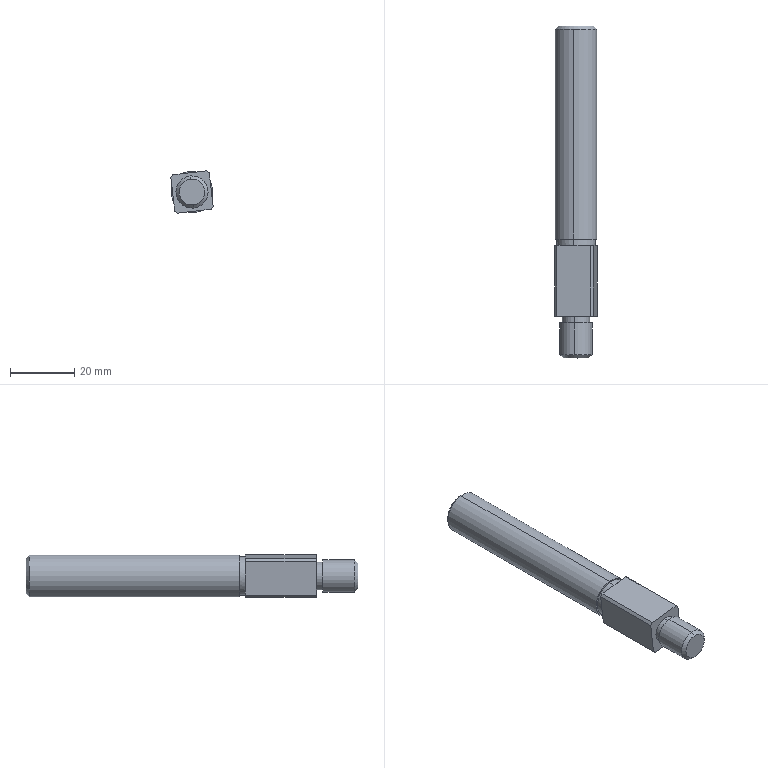Component | SolidWorks | 23-1 | 1 solid | 29 faces | box 13.13 x 103 x 13.13 mm | volume 13082 mm3 | plane 13 | cylinder 12 | cone 4 | commonest cylinder face diameters 16 x4 10 x2 8.5 x2 12 x2 13 x2
STEP:
#1=COLOUR_RGB('',0.7922,0.8196,0.9333);
#2=FILL_AREA_STYLE_COLOUR('',#1);
#3=FILL_AREA_STYLE('',(#2));
#4=SURFACE_STYLE_FILL_AREA(#3);
#5=SURFACE_SIDE_STYLE('',(#4));
#6=SURFACE_STYLE_USAGE(.BOTH.,#5);
#7=PRESENTATION_STYLE_ASSIGNMENT((#6));
#8=CARTESIAN_POINT('',(-5.893,13.153,28.394));
#9=VERTEX_POINT('',#8);
#10=CARTESIAN_POINT('',(-5.843,13.153,27.964));
#11=VERTEX_POINT('',#10);
#12=CARTESIAN_POINT('',(-5.868,13.153,28.179));
#13=DIRECTION('',(0.,1.,-0.));
#14=DIRECTION('',(0.114,0.,-0.9935));
#15=AXIS2_PLACEMENT_3D('',#12,#13,#14);
#16=CIRCLE('',#15,0.2165);
#17=EDGE_CURVE('',#9,#11,#16,.T.);
#18=ORIENTED_EDGE('',*,*,#17,.F.);
#19=CARTESIAN_POINT('',(-5.897,13.114,28.433));
#20=VERTEX_POINT('',#19);
#21=CARTESIAN_POINT('',(-5.897,13.114,28.433));
#22=DIRECTION('',(-0.08059,-0.7071,0.7025));
#23=VECTOR('',#22,39.37);
#24=LINE('',#21,#23);
#25=EDGE_CURVE('',#9,#20,#24,.T.);
#26=ORIENTED_EDGE('',*,*,#25,.T.);
#27=CARTESIAN_POINT('',(-5.839,13.114,27.925));
#28=VERTEX_POINT('',#27);
#29=CARTESIAN_POINT('',(-5.868,13.114,28.179));
#30=DIRECTION('',(-0.,-1.,0.));
#31=DIRECTION('',(0.114,0.,-0.9935));
#32=AXIS2_PLACEMENT_3D('',#29,#30,#31);
#33=CIRCLE('',#32,0.2559);
#34=EDGE_CURVE('',#28,#20,#33,.T.);
#35=ORIENTED_EDGE('',*,*,#34,.F.);
#36=CARTESIAN_POINT('',(-5.839,13.114,27.925));
#37=DIRECTION('',(0.08059,-0.7071,-0.7025));
#38=VECTOR('',#37,39.37);
#39=LINE('',#36,#38);
#40=EDGE_CURVE('',#11,#28,#39,.T.);
#41=ORIENTED_EDGE('',*,*,#40,.F.);
#42=EDGE_LOOP('',(#18,#26,#35,#41));
#43=FACE_OUTER_BOUND('',#42,.T.);
#44=CARTESIAN_POINT('',(-5.868,13.114,28.179));
#45=DIRECTION('',(-0.,-1.,0.));
#46=DIRECTION('',(0.114,0.,-0.9935));
#47=AXIS2_PLACEMENT_3D('',#44,#45,#46);
#48=CONICAL_SURFACE('',#47,0.2559,0.7854);
#49=ADVANCED_FACE('',(#43),#48,.T.);
#50=CARTESIAN_POINT('',(-5.85,9.098,28.023));
#51=VERTEX_POINT('',#50);
#52=CARTESIAN_POINT('',(-5.886,9.098,28.336));
#53=VERTEX_POINT('',#52);
#54=CARTESIAN_POINT('',(-5.868,9.098,28.179));
#55=DIRECTION('',(-0.,-1.,0.));
#56=DIRECTION('',(-0.114,0.,0.9935));
#57=AXIS2_PLACEMENT_3D('',#54,#55,#56);
#58=CIRCLE('',#57,0.1575);
#59=EDGE_CURVE('',#51,#53,#58,.T.);
#60=ORIENTED_EDGE('',*,*,#59,.F.);
#61=CARTESIAN_POINT('',(-5.845,9.137,27.984));
#62=VERTEX_POINT('',#61);
#63=CARTESIAN_POINT('',(-5.85,9.098,28.023));
#64=DIRECTION('',(0.08059,0.7071,-0.7025));
#65=VECTOR('',#64,39.37);
#66=LINE('',#63,#65);
#67=EDGE_CURVE('',#51,#62,#66,.T.);
#68=ORIENTED_EDGE('',*,*,#67,.T.);
#69=CARTESIAN_POINT('',(-5.89,9.137,28.375));
#70=VERTEX_POINT('',#69);
#71=CARTESIAN_POINT('',(-5.868,9.137,28.179));
#72=DIRECTION('',(0.,1.,-0.));
#73=DIRECTION('',(-0.114,0.,0.9935));
#74=AXIS2_PLACEMENT_3D('',#71,#72,#73);
#75=CIRCLE('',#74,0.1969);
#76=EDGE_CURVE('',#70,#62,#75,.T.);
#77=ORIENTED_EDGE('',*,*,#76,.F.);
#78=CARTESIAN_POINT('',(-5.886,9.098,28.336));
#79=DIRECTION('',(-0.08059,0.7071,0.7025));
#80=VECTOR('',#79,39.37);
#81=LINE('',#78,#80);
#82=EDGE_CURVE('',#53,#70,#81,.T.);
#83=ORIENTED_EDGE('',*,*,#82,.F.);
#84=EDGE_LOOP('',(#60,#68,#77,#83));
#85=FACE_OUTER_BOUND('',#84,.T.);
#86=CARTESIAN_POINT('',(-5.868,9.098,28.179));
#87=DIRECTION('',(0.,1.,-0.));
#88=DIRECTION('',(-0.114,0.,0.9935));
#89=AXIS2_PLACEMENT_3D('',#86,#87,#88);
#90=CONICAL_SURFACE('',#89,0.1575,0.7854);
#91=ADVANCED_FACE('',(#85),#90,.T.);
#92=CARTESIAN_POINT('',(-5.845,9.527,27.984));
#93=VERTEX_POINT('',#92);
#94=CARTESIAN_POINT('',(-5.89,9.527,28.375));
#95=VERTEX_POINT('',#94);
#96=CARTESIAN_POINT('',(-5.868,9.527,28.179));
#97=DIRECTION('',(-0.,-1.,0.));
#98=DIRECTION('',(0.114,0.,-0.9935));
#99=AXIS2_PLACEMENT_3D('',#96,#97,#98);
#100=CIRCLE('',#99,0.1969);
#101=EDGE_CURVE('',#93,#95,#100,.T.);
#102=ORIENTED_EDGE('',*,*,#101,.T.);
#103=CARTESIAN_POINT('',(-5.89,9.098,28.375));
#104=DIRECTION('',(-0.,-1.,0.));
#105=VECTOR('',#104,39.37);
#106=LINE('',#103,#105);
#107=EDGE_CURVE('',#95,#70,#106,.T.);
#108=ORIENTED_EDGE('',*,*,#107,.T.);
#109=ORIENTED_EDGE('',*,*,#76,.T.);
#110=CARTESIAN_POINT('',(-5.845,9.098,27.984));
#111=DIRECTION('',(-0.,-1.,0.));
#112=VECTOR('',#111,39.37);
#113=LINE('',#110,#112);
#114=EDGE_CURVE('',#93,#62,#113,.T.);
#115=ORIENTED_EDGE('',*,*,#114,.F.);
#116=EDGE_LOOP('',(#102,#108,#109,#115));
#117=FACE_OUTER_BOUND('',#116,.T.);
#118=CARTESIAN_POINT('',(-5.868,9.098,28.179));
#119=DIRECTION('',(-0.,-1.,0.));
#120=DIRECTION('',(0.114,0.,-0.9935));
#121=AXIS2_PLACEMENT_3D('',#118,#119,#120);
#122=CYLINDRICAL_SURFACE('',#121,0.1969);
#123=ADVANCED_FACE('',(#117),#122,.T.);
#124=CARTESIAN_POINT('',(-5.849,9.606,28.013));
#125=VERTEX_POINT('',#124);
#126=CARTESIAN_POINT('',(-5.887,9.606,28.345));
#127=VERTEX_POINT('',#126);
#128=CARTESIAN_POINT('',(-5.868,9.606,28.179));
#129=DIRECTION('',(-0.,-1.,0.));
#130=DIRECTION('',(0.114,0.,-0.9935));
#131=AXIS2_PLACEMENT_3D('',#128,#129,#130);
#132=CIRCLE('',#131,0.1673);
#133=EDGE_CURVE('',#125,#127,#132,.T.);
#134=ORIENTED_EDGE('',*,*,#133,.T.);
#135=CARTESIAN_POINT('',(-5.887,9.527,28.345));
#136=VERTEX_POINT('',#135);
#137=CARTESIAN_POINT('',(-5.887,9.098,28.345));
#138=DIRECTION('',(-0.,-1.,0.));
#139=VECTOR('',#138,39.37);
#140=LINE('',#137,#139);
#141=EDGE_CURVE('',#127,#136,#140,.T.);
#142=ORIENTED_EDGE('',*,*,#141,.T.);
#143=CARTESIAN_POINT('',(-5.849,9.527,28.013));
#144=VERTEX_POINT('',#143);
#145=CARTESIAN_POINT('',(-5.868,9.527,28.179));
#146=DIRECTION('',(-0.,-1.,0.));
#147=DIRECTION('',(0.114,0.,-0.9935));
#148=AXIS2_PLACEMENT_3D('',#145,#146,#147);
#149=CIRCLE('',#148,0.1673);
#150=EDGE_CURVE('',#144,#136,#149,.T.);
#151=ORIENTED_EDGE('',*,*,#150,.F.);
#152=CARTESIAN_POINT('',(-5.849,9.098,28.013));
#153=DIRECTION('',(-0.,-1.,0.));
#154=VECTOR('',#153,39.37);
#155=LINE('',#152,#154);
#156=EDGE_CURVE('',#125,#144,#155,.T.);
#157=ORIENTED_EDGE('',*,*,#156,.F.);
#158=EDGE_LOOP('',(#134,#142,#151,#157));
#159=FACE_OUTER_BOUND('',#158,.T.);
#160=CARTESIAN_POINT('',(-5.868,9.098,28.179));
#161=DIRECTION('',(-0.,-1.,0.));
#162=DIRECTION('',(0.114,0.,-0.9935));
#163=AXIS2_PLACEMENT_3D('',#160,#161,#162);
#164=CYLINDRICAL_SURFACE('',#163,0.1673);
#165=ADVANCED_FACE('',(#159),#164,.T.);
#166=CARTESIAN_POINT('',(-5.841,10.551,27.944));
#167=VERTEX_POINT('',#166);
#168=CARTESIAN_POINT('',(-5.895,10.551,28.414));
#169=VERTEX_POINT('',#168);
#170=CARTESIAN_POINT('',(-5.868,10.551,28.179));
#171=DIRECTION('',(-0.,-1.,0.));
#172=DIRECTION('',(0.114,0.,-0.9935));
#173=AXIS2_PLACEMENT_3D('',#170,#171,#172);
#174=CIRCLE('',#173,0.2362);
#175=EDGE_CURVE('',#167,#169,#174,.T.);
#176=ORIENTED_EDGE('',*,*,#175,.T.);
#177=CARTESIAN_POINT('',(-5.895,10.472,28.414));
#178=VERTEX_POINT('',#177);
#179=CARTESIAN_POINT('',(-5.895,9.098,28.414));
#180=DIRECTION('',(-0.,-1.,0.));
#181=VECTOR('',#180,39.37);
#182=LINE('',#179,#181);
#183=EDGE_CURVE('',#169,#178,#182,.T.);
#184=ORIENTED_EDGE('',*,*,#183,.T.);
#185=CARTESIAN_POINT('',(-5.633,10.472,28.206));
#186=VERTEX_POINT('',#185);
#187=CARTESIAN_POINT('',(-5.868,10.472,28.179));
#188=DIRECTION('',(-0.,-1.,0.));
#189=DIRECTION('',(0.114,0.,-0.9935));
#190=AXIS2_PLACEMENT_3D('',#187,#188,#189);
#191=CIRCLE('',#190,0.2362);
#192=EDGE_CURVE('',#186,#178,#191,.T.);
#193=ORIENTED_EDGE('',*,*,#192,.F.);
#194=CARTESIAN_POINT('',(-5.841,10.472,27.944));
#195=VERTEX_POINT('',#194);
#196=CARTESIAN_POINT('',(-5.868,10.472,28.179));
#197=DIRECTION('',(-0.,-1.,0.));
#198=DIRECTION('',(0.114,0.,-0.9935));
#199=AXIS2_PLACEMENT_3D('',#196,#197,#198);
#200=CIRCLE('',#199,0.2362);
#201=EDGE_CURVE('',#195,#186,#200,.T.);
#202=ORIENTED_EDGE('',*,*,#201,.F.);
#203=CARTESIAN_POINT('',(-5.841,9.098,27.944));
#204=DIRECTION('',(-0.,-1.,0.));
#205=VECTOR('',#204,39.37);
#206=LINE('',#203,#205);
#207=EDGE_CURVE('',#167,#195,#206,.T.);
#208=ORIENTED_EDGE('',*,*,#207,.F.);
#209=EDGE_LOOP('',(#176,#184,#193,#202,#208));
#210=FACE_OUTER_BOUND('',#209,.T.);
#211=CARTESIAN_POINT('',(-5.868,9.098,28.179));
#212=DIRECTION('',(-0.,-1.,0.));
#213=DIRECTION('',(0.114,0.,-0.9935));
#214=AXIS2_PLACEMENT_3D('',#211,#212,#213);
#215=CYLINDRICAL_SURFACE('',#214,0.2362);
#216=ADVANCED_FACE('',(#210),#215,.T.);
#217=ORIENTED_EDGE('',*,*,#34,.T.);
#218=CARTESIAN_POINT('',(-5.897,10.551,28.433));
#219=VERTEX_POINT('',#218);
#220=CARTESIAN_POINT('',(-5.897,9.098,28.433));
#221=DIRECTION('',(-0.,-1.,0.));
#222=VECTOR('',#221,39.37);
#223=LINE('',#220,#222);
#224=EDGE_CURVE('',#20,#219,#223,.T.);
#225=ORIENTED_EDGE('',*,*,#224,.T.);
#226=CARTESIAN_POINT('',(-5.839,10.551,27.925));
#227=VERTEX_POINT('',#226);
#228=CARTESIAN_POINT('',(-5.868,10.551,28.179));
#229=DIRECTION('',(-0.,-1.,0.));
#230=DIRECTION('',(0.114,0.,-0.9935));
#231=AXIS2_PLACEMENT_3D('',#228,#229,#230);
#232=CIRCLE('',#231,0.2559);
#233=EDGE_CURVE('',#227,#219,#232,.T.);
#234=ORIENTED_EDGE('',*,*,#233,.F.);
#235=CARTESIAN_POINT('',(-5.839,9.098,27.925));
#236=DIRECTION('',(-0.,-1.,0.));
#237=VECTOR('',#236,39.37);
#238=LINE('',#235,#237);
#239=EDGE_CURVE('',#28,#227,#238,.T.);
#240=ORIENTED_EDGE('',*,*,#239,.F.);
#241=EDGE_LOOP('',(#217,#225,#234,#240));
#242=FACE_OUTER_BOUND('',#241,.T.);
#243=CARTESIAN_POINT('',(-5.868,9.098,28.179));
#244=DIRECTION('',(-0.,-1.,0.));
#245=DIRECTION('',(0.114,0.,-0.9935));
#246=AXIS2_PLACEMENT_3D('',#243,#244,#245);
#247=CYLINDRICAL_SURFACE('',#246,0.2559);
#248=ADVANCED_FACE('',(#242),#247,.T.);
#249=CARTESIAN_POINT('',(-6.102,10.472,28.39));
#250=VERTEX_POINT('',#249);
#251=CARTESIAN_POINT('',(-6.126,10.472,28.359));
#252=VERTEX_POINT('',#251);
#253=CARTESIAN_POINT('',(-5.868,10.472,28.179));
#254=DIRECTION('',(-0.,-1.,0.));
#255=DIRECTION('',(0.114,0.,-0.9935));
#256=AXIS2_PLACEMENT_3D('',#253,#254,#255);
#257=CIRCLE('',#256,0.315);
#258=EDGE_CURVE('',#250,#252,#257,.T.);
#259=ORIENTED_EDGE('',*,*,#258,.F.);
#260=CARTESIAN_POINT('',(-5.895,10.472,28.414));
#261=DIRECTION('',(0.9935,-0.,0.114));
#262=VECTOR('',#261,39.37);
#263=LINE('',#260,#262);
#264=EDGE_CURVE('',#250,#178,#263,.T.);
#265=ORIENTED_EDGE('',*,*,#264,.T.);
#266=CARTESIAN_POINT('',(-6.103,10.472,28.152));
#267=VERTEX_POINT('',#266);
#268=CARTESIAN_POINT('',(-5.868,10.472,28.179));
#269=DIRECTION('',(-0.,-1.,0.));
#270=DIRECTION('',(0.114,0.,-0.9935));
#271=AXIS2_PLACEMENT_3D('',#268,#269,#270);
#272=CIRCLE('',#271,0.2362);
#273=EDGE_CURVE('',#178,#267,#272,.T.);
#274=ORIENTED_EDGE('',*,*,#273,.T.);
#275=CARTESIAN_POINT('',(-6.103,10.472,28.152));
#276=DIRECTION('',(0.114,-0.,-0.9935));
#277=VECTOR('',#276,39.37);
#278=LINE('',#275,#277);
#279=EDGE_CURVE('',#252,#267,#278,.T.);
#280=ORIENTED_EDGE('',*,*,#279,.F.);
#281=EDGE_LOOP('',(#259,#265,#274,#280));
#282=FACE_OUTER_BOUND('',#281,.T.);
#283=CARTESIAN_POINT('',(-5.895,10.472,28.414));
#284=DIRECTION('',(-0.,-1.,0.));
#285=DIRECTION('',(0.114,-0.,-0.9935));
#286=AXIS2_PLACEMENT_3D('',#283,#284,#285);
#287=PLANE('',#286);
#288=ADVANCED_FACE('',(#282),#287,.F.);
#289=ORIENTED_EDGE('',*,*,#192,.T.);
#290=CARTESIAN_POINT('',(-5.688,10.472,28.438));
#291=VERTEX_POINT('',#290);
#292=CARTESIAN_POINT('',(-5.895,10.472,28.414));
#293=DIRECTION('',(0.9935,-0.,0.114));
#294=VECTOR('',#293,39.37);
#295=LINE('',#292,#294);
#296=EDGE_CURVE('',#178,#291,#295,.T.);
#297=ORIENTED_EDGE('',*,*,#296,.T.);
#298=CARTESIAN_POINT('',(-5.657,10.472,28.413));
#299=VERTEX_POINT('',#298);
#300=CARTESIAN_POINT('',(-5.868,10.472,28.179));
#301=DIRECTION('',(-0.,-1.,0.));
#302=DIRECTION('',(0.114,0.,-0.9935));
#303=AXIS2_PLACEMENT_3D('',#300,#301,#302);
#304=CIRCLE('',#303,0.315);
#305=EDGE_CURVE('',#299,#291,#304,.T.);
#306=ORIENTED_EDGE('',*,*,#305,.F.);
#307=CARTESIAN_POINT('',(-5.633,10.472,28.206));
#308=DIRECTION('',(0.114,-0.,-0.9935));
#309=VECTOR('',#308,39.37);
#310=LINE('',#307,#309);
#311=EDGE_CURVE('',#299,#186,#310,.T.);
#312=ORIENTED_EDGE('',*,*,#311,.T.);
#313=EDGE_LOOP('',(#289,#297,#306,#312));
#314=FACE_OUTER_BOUND('',#313,.T.);
#315=CARTESIAN_POINT('',(-5.895,10.472,28.414));
#316=DIRECTION('',(-0.,-1.,0.));
#317=DIRECTION('',(0.114,-0.,-0.9935));
#318=AXIS2_PLACEMENT_3D('',#315,#316,#317);
#319=PLANE('',#318);
#320=ADVANCED_FACE('',(#314),#319,.F.);
#321=CARTESIAN_POINT('',(-6.048,10.472,27.921));
#322=VERTEX_POINT('',#321);
#323=CARTESIAN_POINT('',(-5.841,10.472,27.944));
#324=DIRECTION('',(0.9935,-0.,0.114));
#325=VECTOR('',#324,39.37);
#326=LINE('',#323,#325);
#327=EDGE_CURVE('',#322,#195,#326,.T.);
#328=ORIENTED_EDGE('',*,*,#327,.F.);
#329=CARTESIAN_POINT('',(-6.079,10.472,27.945));
#330=VERTEX_POINT('',#329);
#331=CARTESIAN_POINT('',(-5.868,10.472,28.179));
#332=DIRECTION('',(-0.,-1.,0.));
#333=DIRECTION('',(0.114,0.,-0.9935));
#334=AXIS2_PLACEMENT_3D('',#331,#332,#333);
#335=CIRCLE('',#334,0.315);
#336=EDGE_CURVE('',#330,#322,#335,.T.);
#337=ORIENTED_EDGE('',*,*,#336,.F.);
#338=CARTESIAN_POINT('',(-6.103,10.472,28.152));
#339=DIRECTION('',(0.114,-0.,-0.9935));
#340=VECTOR('',#339,39.37);
#341=LINE('',#338,#340);
#342=EDGE_CURVE('',#267,#330,#341,.T.);
#343=ORIENTED_EDGE('',*,*,#342,.F.);
#344=CARTESIAN_POINT('',(-5.868,10.472,28.179));
#345=DIRECTION('',(-0.,-1.,0.));
#346=DIRECTION('',(0.114,0.,-0.9935));
#347=AXIS2_PLACEMENT_3D('',#344,#345,#346);
#348=CIRCLE('',#347,0.2362);
#349=EDGE_CURVE('',#267,#195,#348,.T.);
#350=ORIENTED_EDGE('',*,*,#349,.T.);
#351=EDGE_LOOP('',(#328,#337,#343,#350));
#352=FACE_OUTER_BOUND('',#351,.T.);
#353=CARTESIAN_POINT('',(-5.895,10.472,28.414));
#354=DIRECTION('',(-0.,-1.,0.));
#355=DIRECTION('',(0.114,-0.,-0.9935));
#356=AXIS2_PLACEMENT_3D('',#353,#354,#355);
#357=PLANE('',#356);
#358=ADVANCED_FACE('',(#352),#357,.F.);
#359=ORIENTED_EDGE('',*,*,#201,.T.);
#360=CARTESIAN_POINT('',(-5.609,10.472,27.999));
#361=VERTEX_POINT('',#360);
#362=CARTESIAN_POINT('',(-5.633,10.472,28.206));
#363=DIRECTION('',(0.114,-0.,-0.9935));
#364=VECTOR('',#363,39.37);
#365=LINE('',#362,#364);
#366=EDGE_CURVE('',#186,#361,#365,.T.);
#367=ORIENTED_EDGE('',*,*,#366,.T.);
#368=CARTESIAN_POINT('',(-5.634,10.472,27.968));
#369=VERTEX_POINT('',#368);
#370=CARTESIAN_POINT('',(-5.868,10.472,28.179));
#371=DIRECTION('',(-0.,-1.,0.));
#372=DIRECTION('',(0.114,0.,-0.9935));
#373=AXIS2_PLACEMENT_3D('',#370,#371,#372);
#374=CIRCLE('',#373,0.315);
#375=EDGE_CURVE('',#369,#361,#374,.T.);
#376=ORIENTED_EDGE('',*,*,#375,.F.);
#377=CARTESIAN_POINT('',(-5.841,10.472,27.944));
#378=DIRECTION('',(0.9935,-0.,0.114));
#379=VECTOR('',#378,39.37);
#380=LINE('',#377,#379);
#381=EDGE_CURVE('',#195,#369,#380,.T.);
#382=ORIENTED_EDGE('',*,*,#381,.F.);
#383=EDGE_LOOP('',(#359,#367,#376,#382));
#384=FACE_OUTER_BOUND('',#383,.T.);
#385=CARTESIAN_POINT('',(-5.895,10.472,28.414));
#386=DIRECTION('',(-0.,-1.,0.));
#387=DIRECTION('',(0.114,-0.,-0.9935));
#388=AXIS2_PLACEMENT_3D('',#385,#386,#387);
#389=PLANE('',#388);
#390=ADVANCED_FACE('',(#384),#389,.F.);
#391=ORIENTED_EDGE('',*,*,#305,.T.);
#392=CARTESIAN_POINT('',(-5.688,9.606,28.438));
#393=VERTEX_POINT('',#392);
#394=CARTESIAN_POINT('',(-5.688,10.472,28.438));
#395=DIRECTION('',(-0.,-1.,0.));
#396=VECTOR('',#395,39.37);
#397=LINE('',#394,#396);
#398=EDGE_CURVE('',#291,#393,#397,.T.);
#399=ORIENTED_EDGE('',*,*,#398,.T.);
#400=CARTESIAN_POINT('',(-5.657,9.606,28.413));
#401=VERTEX_POINT('',#400);
#402=CARTESIAN_POINT('',(-5.868,9.606,28.179));
#403=DIRECTION('',(-0.,-1.,0.));
#404=DIRECTION('',(0.114,0.,-0.9935));
#405=AXIS2_PLACEMENT_3D('',#402,#403,#404);
#406=CIRCLE('',#405,0.315);
#407=EDGE_CURVE('',#401,#393,#406,.T.);
#408=ORIENTED_EDGE('',*,*,#407,.F.);
#409=CARTESIAN_POINT('',(-5.657,10.472,28.413));
#410=DIRECTION('',(-0.,-1.,0.));
#411=VECTOR('',#410,39.37);
#412=LINE('',#409,#411);
#413=EDGE_CURVE('',#299,#401,#412,.T.);
#414=ORIENTED_EDGE('',*,*,#413,.F.);
#415=EDGE_LOOP('',(#391,#399,#408,#414));
#416=FACE_OUTER_BOUND('',#415,.T.);
#417=CARTESIAN_POINT('',(-5.868,9.098,28.179));
#418=DIRECTION('',(-0.,-1.,0.));
#419=DIRECTION('',(0.114,0.,-0.9935));
#420=AXIS2_PLACEMENT_3D('',#417,#418,#419);
#421=CYLINDRICAL_SURFACE('',#420,0.315);
#422=ADVANCED_FACE('',(#416),#421,.T.);
#423=ORIENTED_EDGE('',*,*,#375,.T.);
#424=CARTESIAN_POINT('',(-5.609,9.606,27.999));
#425=VERTEX_POINT('',#424);
#426=CARTESIAN_POINT('',(-5.609,10.472,27.999));
#427=DIRECTION('',(-0.,-1.,0.));
#428=VECTOR('',#427,39.37);
#429=LINE('',#426,#428);
#430=EDGE_CURVE('',#361,#425,#429,.T.);
#431=ORIENTED_EDGE('',*,*,#430,.T.);
#432=CARTESIAN_POINT('',(-5.634,9.606,27.968));
#433=VERTEX_POINT('',#432);
#434=CARTESIAN_POINT('',(-5.868,9.606,28.179));
#435=DIRECTION('',(-0.,-1.,0.));
#436=DIRECTION('',(0.114,0.,-0.9935));
#437=AXIS2_PLACEMENT_3D('',#434,#435,#436);
#438=CIRCLE('',#437,0.315);
#439=EDGE_CURVE('',#433,#425,#438,.T.);
#440=ORIENTED_EDGE('',*,*,#439,.F.);
#441=CARTESIAN_POINT('',(-5.634,10.472,27.968));
#442=DIRECTION('',(-0.,-1.,0.));
#443=VECTOR('',#442,39.37);
#444=LINE('',#441,#443);
#445=EDGE_CURVE('',#369,#433,#444,.T.);
#446=ORIENTED_EDGE('',*,*,#445,.F.);
#447=EDGE_LOOP('',(#423,#431,#440,#446));
#448=FACE_OUTER_BOUND('',#447,.T.);
#449=CARTESIAN_POINT('',(-5.868,9.098,28.179));
#450=DIRECTION('',(-0.,-1.,0.));
#451=DIRECTION('',(0.114,0.,-0.9935));
#452=AXIS2_PLACEMENT_3D('',#449,#450,#451);
#453=CYLINDRICAL_SURFACE('',#452,0.315);
#454=ADVANCED_FACE('',(#448),#453,.T.);
#455=CARTESIAN_POINT('',(-6.102,9.606,28.39));
#456=VERTEX_POINT('',#455);
#457=CARTESIAN_POINT('',(-6.126,9.606,28.359));
#458=VERTEX_POINT('',#457);
#459=CARTESIAN_POINT('',(-5.868,9.606,28.179));
#460=DIRECTION('',(-0.,-1.,0.));
#461=DIRECTION('',(0.114,0.,-0.9935));
#462=AXIS2_PLACEMENT_3D('',#459,#460,#461);
#463=CIRCLE('',#462,0.315);
#464=EDGE_CURVE('',#456,#458,#463,.T.);
#465=ORIENTED_EDGE('',*,*,#464,.F.);
#466=CARTESIAN_POINT('',(-6.102,10.472,28.39));
#467=DIRECTION('',(-0.,-1.,0.));
#468=VECTOR('',#467,39.37);
#469=LINE('',#466,#468);
#470=EDGE_CURVE('',#250,#456,#469,.T.);
#471=ORIENTED_EDGE('',*,*,#470,.F.);
#472=ORIENTED_EDGE('',*,*,#258,.T.);
#473=CARTESIAN_POINT('',(-6.126,10.472,28.359));
#474=DIRECTION('',(-0.,-1.,0.));
#475=VECTOR('',#474,39.37);
#476=LINE('',#473,#475);
#477=EDGE_CURVE('',#252,#458,#476,.T.);
#478=ORIENTED_EDGE('',*,*,#477,.T.);
#479=EDGE_LOOP('',(#465,#471,#472,#478));
#480=FACE_OUTER_BOUND('',#479,.T.);
#481=CARTESIAN_POINT('',(-5.868,9.098,28.179));
#482=DIRECTION('',(-0.,-1.,0.));
#483=DIRECTION('',(0.114,0.,-0.9935));
#484=AXIS2_PLACEMENT_3D('',#481,#482,#483);
#485=CYLINDRICAL_SURFACE('',#484,0.315);
#486=ADVANCED_FACE('',(#480),#485,.T.);
#487=CARTESIAN_POINT('',(-6.048,9.606,27.921));
#488=VERTEX_POINT('',#487);
#489=CARTESIAN_POINT('',(-6.048,10.472,27.921));
#490=DIRECTION('',(-0.,-1.,0.));
#491=VECTOR('',#490,39.37);
#492=LINE('',#489,#491);
#493=EDGE_CURVE('',#322,#488,#492,.T.);
#494=ORIENTED_EDGE('',*,*,#493,.T.);
#495=CARTESIAN_POINT('',(-6.079,9.606,27.945));
#496=VERTEX_POINT('',#495);
#497=CARTESIAN_POINT('',(-5.868,9.606,28.179));
#498=DIRECTION('',(-0.,-1.,0.));
#499=DIRECTION('',(0.114,0.,-0.9935));
#500=AXIS2_PLACEMENT_3D('',#497,#498,#499);
#501=CIRCLE('',#500,0.315);
#502=EDGE_CURVE('',#496,#488,#501,.T.);
#503=ORIENTED_EDGE('',*,*,#502,.F.);
#504=CARTESIAN_POINT('',(-6.079,10.472,27.945));
#505=DIRECTION('',(-0.,-1.,0.));
#506=VECTOR('',#505,39.37);
#507=LINE('',#504,#506);
#508=EDGE_CURVE('',#330,#496,#507,.T.);
#509=ORIENTED_EDGE('',*,*,#508,.F.);
#510=ORIENTED_EDGE('',*,*,#336,.T.);
#511=EDGE_LOOP('',(#494,#503,#509,#510));
#512=FACE_OUTER_BOUND('',#511,.T.);
#513=CARTESIAN_POINT('',(-5.868,9.098,28.179));
#514=DIRECTION('',(-0.,-1.,0.));
#515=DIRECTION('',(0.114,0.,-0.9935));
#516=AXIS2_PLACEMENT_3D('',#513,#514,#515);
#517=CYLINDRICAL_SURFACE('',#516,0.315);
#518=ADVANCED_FACE('',(#512),#517,.T.);
#519=ORIENTED_EDGE('',*,*,#133,.F.);
#520=CARTESIAN_POINT('',(-5.868,9.606,28.179));
#521=DIRECTION('',(-0.,-1.,0.));
#522=DIRECTION('',(0.114,0.,-0.9935));
#523=AXIS2_PLACEMENT_3D('',#520,#521,#522);
#524=CIRCLE('',#523,0.1673);
#525=EDGE_CURVE('',#127,#125,#524,.T.);
#526=ORIENTED_EDGE('',*,*,#525,.F.);
#527=EDGE_LOOP('',(#519,#526));
#528=FACE_BOUND('',#527,.T.);
#529=ORIENTED_EDGE('',*,*,#407,.T.);
#530=CARTESIAN_POINT('',(-5.895,9.606,28.414));
#531=DIRECTION('',(0.9935,-0.,0.114));
#532=VECTOR('',#531,39.37);
#533=LINE('',#530,#532);
#534=EDGE_CURVE('',#456,#393,#533,.T.);
#535=ORIENTED_EDGE('',*,*,#534,.F.);
#536=ORIENTED_EDGE('',*,*,#464,.T.);
#537=CARTESIAN_POINT('',(-6.103,9.606,28.152));
#538=DIRECTION('',(0.114,-0.,-0.9935));
#539=VECTOR('',#538,39.37);
#540=LINE('',#537,#539);
#541=EDGE_CURVE('',#458,#496,#540,.T.);
#542=ORIENTED_EDGE('',*,*,#541,.T.);
#543=ORIENTED_EDGE('',*,*,#502,.T.);
#544=CARTESIAN_POINT('',(-5.841,9.606,27.944));
#545=DIRECTION('',(0.9935,-0.,0.114));
#546=VECTOR('',#545,39.37);
#547=LINE('',#544,#546);
#548=EDGE_CURVE('',#488,#433,#547,.T.);
#549=ORIENTED_EDGE('',*,*,#548,.T.);
#550=ORIENTED_EDGE('',*,*,#439,.T.);
#551=CARTESIAN_POINT('',(-5.633,9.606,28.206));
#552=DIRECTION('',(0.114,-0.,-0.9935));
#553=VECTOR('',#552,39.37);
#554=LINE('',#551,#553);
#555=EDGE_CURVE('',#401,#425,#554,.T.);
#556=ORIENTED_EDGE('',*,*,#555,.F.);
#557=EDGE_LOOP('',(#529,#535,#536,#542,#543,#549,#550,#556));
#558=FACE_OUTER_BOUND('',#557,.T.);
#559=CARTESIAN_POINT('',(-5.904,9.606,28.492));
#560=DIRECTION('',(0.,1.,-0.));
#561=DIRECTION('',(-0.114,0.,0.9935));
#562=AXIS2_PLACEMENT_3D('',#559,#560,#561);
#563=PLANE('',#562);
#564=ADVANCED_FACE('',(#528,#558),#563,.F.);
#565=CARTESIAN_POINT('',(-5.868,9.098,28.179));
#566=DIRECTION('',(-0.,-1.,0.));
#567=DIRECTION('',(-0.114,0.,0.9935));
#568=AXIS2_PLACEMENT_3D('',#565,#566,#567);
#569=CIRCLE('',#568,0.1575);
#570=EDGE_CURVE('',#53,#51,#569,.T.);
#571=ORIENTED_EDGE('',*,*,#570,.T.);
#572=ORIENTED_EDGE('',*,*,#59,.T.);
#573=EDGE_LOOP('',(#571,#572));
#574=FACE_OUTER_BOUND('',#573,.T.);
#575=CARTESIAN_POINT('',(-5.89,9.098,28.375));
#576=DIRECTION('',(0.,1.,-0.));
#577=DIRECTION('',(-0.114,0.,0.9935));
#578=AXIS2_PLACEMENT_3D('',#575,#576,#577);
#579=PLANE('',#578);
#580=ADVANCED_FACE('',(#574),#579,.F.);
#581=CARTESIAN_POINT('',(-5.868,13.153,28.179));
#582=DIRECTION('',(0.,1.,-0.));
#583=DIRECTION('',(0.114,0.,-0.9935));
#584=AXIS2_PLACEMENT_3D('',#581,#582,#583);
#585=CIRCLE('',#584,0.2165);
#586=EDGE_CURVE('',#11,#9,#585,.T.);
#587=ORIENTED_EDGE('',*,*,#586,.T.);
#588=ORIENTED_EDGE('',*,*,#17,.T.);
#589=EDGE_LOOP('',(#587,#588));
#590=FACE_OUTER_BOUND('',#589,.T.);
#591=CARTESIAN_POINT('',(-5.868,13.153,28.179));
#592=DIRECTION('',(-0.,-1.,0.));
#593=DIRECTION('',(0.114,-0.,-0.9935));
#594=AXIS2_PLACEMENT_3D('',#591,#592,#593);
#595=PLANE('',#594);
#596=ADVANCED_FACE('',(#590),#595,.F.);
#597=ORIENTED_EDGE('',*,*,#224,.F.);
#598=CARTESIAN_POINT('',(-5.868,13.114,28.179));
#599=DIRECTION('',(-0.,-1.,0.));
#600=DIRECTION('',(0.114,0.,-0.9935));
#601=AXIS2_PLACEMENT_3D('',#598,#599,#600);
#602=CIRCLE('',#601,0.2559);
#603=EDGE_CURVE('',#20,#28,#602,.T.);
#604=ORIENTED_EDGE('',*,*,#603,.T.);
#605=ORIENTED_EDGE('',*,*,#239,.T.);
#606=CARTESIAN_POINT('',(-5.868,10.551,28.179));
#607=DIRECTION('',(-0.,-1.,0.));
#608=DIRECTION('',(0.114,0.,-0.9935));
#609=AXIS2_PLACEMENT_3D('',#606,#607,#608);
#610=CIRCLE('',#609,0.2559);
#611=EDGE_CURVE('',#219,#227,#610,.T.);
#612=ORIENTED_EDGE('',*,*,#611,.F.);
#613=EDGE_LOOP('',(#597,#604,#605,#612));
#614=FACE_OUTER_BOUND('',#613,.T.);
#615=CARTESIAN_POINT('',(-5.868,9.098,28.179));
#616=DIRECTION('',(-0.,-1.,0.));
#617=DIRECTION('',(0.114,0.,-0.9935));
#618=AXIS2_PLACEMENT_3D('',#615,#616,#617);
#619=CYLINDRICAL_SURFACE('',#618,0.2559);
#620=ADVANCED_FACE('',(#614),#619,.T.);
#621=ORIENTED_EDGE('',*,*,#175,.F.);
#622=CARTESIAN_POINT('',(-5.868,10.551,28.179));
#623=DIRECTION('',(-0.,-1.,0.));
#624=DIRECTION('',(0.114,0.,-0.9935));
#625=AXIS2_PLACEMENT_3D('',#622,#623,#624);
#626=CIRCLE('',#625,0.2362);
#627=EDGE_CURVE('',#169,#167,#626,.T.);
#628=ORIENTED_EDGE('',*,*,#627,.F.);
#629=EDGE_LOOP('',(#621,#628));
#630=FACE_BOUND('',#629,.T.);
#631=ORIENTED_EDGE('',*,*,#233,.T.);
#632=ORIENTED_EDGE('',*,*,#611,.T.);
#633=EDGE_LOOP('',(#631,#632));
#634=FACE_OUTER_BOUND('',#633,.T.);
#635=CARTESIAN_POINT('',(-5.897,10.551,28.433));
#636=DIRECTION('',(0.,1.,-0.));
#637=DIRECTION('',(-0.114,0.,0.9935));
#638=AXIS2_PLACEMENT_3D('',#635,#636,#637);
#639=PLANE('',#638);
#640=ADVANCED_FACE('',(#630,#634),#639,.F.);
#641=ORIENTED_EDGE('',*,*,#183,.F.);
#642=ORIENTED_EDGE('',*,*,#627,.T.);
#643=ORIENTED_EDGE('',*,*,#207,.T.);
#644=ORIENTED_EDGE('',*,*,#349,.F.);
#645=ORIENTED_EDGE('',*,*,#273,.F.);
#646=EDGE_LOOP('',(#641,#642,#643,#644,#645));
#647=FACE_OUTER_BOUND('',#646,.T.);
#648=CARTESIAN_POINT('',(-5.868,9.098,28.179));
#649=DIRECTION('',(-0.,-1.,0.));
#650=DIRECTION('',(0.114,0.,-0.9935));
#651=AXIS2_PLACEMENT_3D('',#648,#649,#650);
#652=CYLINDRICAL_SURFACE('',#651,0.2362);
#653=ADVANCED_FACE('',(#647),#652,.T.);
#654=ORIENTED_EDGE('',*,*,#141,.F.);
#655=ORIENTED_EDGE('',*,*,#525,.T.);
#656=ORIENTED_EDGE('',*,*,#156,.T.);
#657=CARTESIAN_POINT('',(-5.868,9.527,28.179));
#658=DIRECTION('',(-0.,-1.,0.));
#659=DIRECTION('',(0.114,0.,-0.9935));
#660=AXIS2_PLACEMENT_3D('',#657,#658,#659);
#661=CIRCLE('',#660,0.1673);
#662=EDGE_CURVE('',#136,#144,#661,.T.);
#663=ORIENTED_EDGE('',*,*,#662,.F.);
#664=EDGE_LOOP('',(#654,#655,#656,#663));
#665=FACE_OUTER_BOUND('',#664,.T.);
#666=CARTESIAN_POINT('',(-5.868,9.098,28.179));
#667=DIRECTION('',(-0.,-1.,0.));
#668=DIRECTION('',(0.114,0.,-0.9935));
#669=AXIS2_PLACEMENT_3D('',#666,#667,#668);
#670=CYLINDRICAL_SURFACE('',#669,0.1673);
#671=ADVANCED_FACE('',(#665),#670,.T.);
#672=ORIENTED_EDGE('',*,*,#101,.F.);
#673=CARTESIAN_POINT('',(-5.868,9.527,28.179));
#674=DIRECTION('',(-0.,-1.,0.));
#675=DIRECTION('',(0.114,0.,-0.9935));
#676=AXIS2_PLACEMENT_3D('',#673,#674,#675);
#677=CIRCLE('',#676,0.1969);
#678=EDGE_CURVE('',#95,#93,#677,.T.);
#679=ORIENTED_EDGE('',*,*,#678,.F.);
#680=EDGE_LOOP('',(#672,#679));
#681=FACE_OUTER_BOUND('',#680,.T.);
#682=ORIENTED_EDGE('',*,*,#150,.T.);
#683=ORIENTED_EDGE('',*,*,#662,.T.);
#684=EDGE_LOOP('',(#682,#683));
#685=FACE_BOUND('',#684,.T.);
#686=CARTESIAN_POINT('',(-5.887,9.527,28.345));
#687=DIRECTION('',(-0.,-1.,0.));
#688=DIRECTION('',(0.114,-0.,-0.9935));
#689=AXIS2_PLACEMENT_3D('',#686,#687,#688);
#690=PLANE('',#689);
#691=ADVANCED_FACE('',(#681,#685),#690,.F.);
#692=ORIENTED_EDGE('',*,*,#107,.F.);
#693=ORIENTED_EDGE('',*,*,#678,.T.);
#694=ORIENTED_EDGE('',*,*,#114,.T.);
#695=CARTESIAN_POINT('',(-5.868,9.137,28.179));
#696=DIRECTION('',(0.,1.,-0.));
#697=DIRECTION('',(-0.114,0.,0.9935));
#698=AXIS2_PLACEMENT_3D('',#695,#696,#697);
#699=CIRCLE('',#698,0.1969);
#700=EDGE_CURVE('',#62,#70,#699,.T.);
#701=ORIENTED_EDGE('',*,*,#700,.T.);
#702=EDGE_LOOP('',(#692,#693,#694,#701));
#703=FACE_OUTER_BOUND('',#702,.T.);
#704=CARTESIAN_POINT('',(-5.868,9.098,28.179));
#705=DIRECTION('',(-0.,-1.,0.));
#706=DIRECTION('',(0.114,0.,-0.9935));
#707=AXIS2_PLACEMENT_3D('',#704,#705,#706);
#708=CYLINDRICAL_SURFACE('',#707,0.1969);
#709=ADVANCED_FACE('',(#703),#708,.T.);
#710=ORIENTED_EDGE('',*,*,#67,.F.);
#711=ORIENTED_EDGE('',*,*,#570,.F.);
#712=ORIENTED_EDGE('',*,*,#82,.T.);
#713=ORIENTED_EDGE('',*,*,#700,.F.);
#714=EDGE_LOOP('',(#710,#711,#712,#713));
#715=FACE_OUTER_BOUND('',#714,.T.);
#716=CARTESIAN_POINT('',(-5.868,9.098,28.179));
#717=DIRECTION('',(0.,1.,-0.));
#718=DIRECTION('',(-0.114,0.,0.9935));
#719=AXIS2_PLACEMENT_3D('',#716,#717,#718);
#720=CONICAL_SURFACE('',#719,0.1575,0.7854);
#721=ADVANCED_FACE('',(#715),#720,.T.);
#722=ORIENTED_EDGE('',*,*,#25,.F.);
#723=ORIENTED_EDGE('',*,*,#586,.F.);
#724=ORIENTED_EDGE('',*,*,#40,.T.);
#725=ORIENTED_EDGE('',*,*,#603,.F.);
#726=EDGE_LOOP('',(#722,#723,#724,#725));
#727=FACE_OUTER_BOUND('',#726,.T.);
#728=CARTESIAN_POINT('',(-5.868,13.114,28.179));
#729=DIRECTION('',(-0.,-1.,0.));
#730=DIRECTION('',(0.114,0.,-0.9935));
#731=AXIS2_PLACEMENT_3D('',#728,#729,#730);
#732=CONICAL_SURFACE('',#731,0.2559,0.7854);
#733=ADVANCED_FACE('',(#727),#732,.T.);
#734=ORIENTED_EDGE('',*,*,#541,.F.);
#735=ORIENTED_EDGE('',*,*,#477,.F.);
#736=ORIENTED_EDGE('',*,*,#279,.T.);
#737=ORIENTED_EDGE('',*,*,#342,.T.);
#738=ORIENTED_EDGE('',*,*,#508,.T.);
#739=EDGE_LOOP('',(#734,#735,#736,#737,#738));
#740=FACE_OUTER_BOUND('',#739,.T.);
#741=CARTESIAN_POINT('',(-6.103,10.472,28.152));
#742=DIRECTION('',(-0.9935,0.,-0.114));
#743=DIRECTION('',(-0.114,0.,0.9935));
#744=AXIS2_PLACEMENT_3D('',#741,#742,#743);
#745=PLANE('',#744);
#746=ADVANCED_FACE('',(#740),#745,.T.);
#747=ORIENTED_EDGE('',*,*,#548,.F.);
#748=ORIENTED_EDGE('',*,*,#493,.F.);
#749=ORIENTED_EDGE('',*,*,#327,.T.);
#750=ORIENTED_EDGE('',*,*,#381,.T.);
#751=ORIENTED_EDGE('',*,*,#445,.T.);
#752=EDGE_LOOP('',(#747,#748,#749,#750,#751));
#753=FACE_OUTER_BOUND('',#752,.T.);
#754=CARTESIAN_POINT('',(-5.841,10.472,27.944));
#755=DIRECTION('',(0.114,-0.,-0.9935));
#756=DIRECTION('',(0.,1.,-0.));
#757=AXIS2_PLACEMENT_3D('',#754,#755,#756);
#758=PLANE('',#757);
#759=ADVANCED_FACE('',(#753),#758,.T.);
#760=ORIENTED_EDGE('',*,*,#555,.T.);
#761=ORIENTED_EDGE('',*,*,#430,.F.);
#762=ORIENTED_EDGE('',*,*,#366,.F.);
#763=ORIENTED_EDGE('',*,*,#311,.F.);
#764=ORIENTED_EDGE('',*,*,#413,.T.);
#765=EDGE_LOOP('',(#760,#761,#762,#763,#764));
#766=FACE_OUTER_BOUND('',#765,.T.);
#767=CARTESIAN_POINT('',(-5.633,10.472,28.206));
#768=DIRECTION('',(-0.9935,0.,-0.114));
#769=DIRECTION('',(-0.114,0.,0.9935));
#770=AXIS2_PLACEMENT_3D('',#767,#768,#769);
#771=PLANE('',#770);
#772=ADVANCED_FACE('',(#766),#771,.F.);
#773=ORIENTED_EDGE('',*,*,#534,.T.);
#774=ORIENTED_EDGE('',*,*,#398,.F.);
#775=ORIENTED_EDGE('',*,*,#296,.F.);
#776=ORIENTED_EDGE('',*,*,#264,.F.);
#777=ORIENTED_EDGE('',*,*,#470,.T.);
#778=EDGE_LOOP('',(#773,#774,#775,#776,#777));
#779=FACE_OUTER_BOUND('',#778,.T.);
#780=CARTESIAN_POINT('',(-5.895,10.472,28.414));
#781=DIRECTION('',(0.114,-0.,-0.9935));
#782=DIRECTION('',(0.,1.,-0.));
#783=AXIS2_PLACEMENT_3D('',#780,#781,#782);
#784=PLANE('',#783);
#785=ADVANCED_FACE('',(#779),#784,.F.);
#786=CLOSED_SHELL('',(#49,#91,#123,#165,#216,#248,#288,#320,#358,#390,#422,#454,#486,#518,#564,#580,#596,#620,#640,#653,#671,#691,#709,#721,#733,#746,#759,#772,#785));
#787=MANIFOLD_SOLID_BREP('',#786);
#788=STYLED_ITEM('',(#7),#787);
#789=PRESENTATION_LAYER_ASSIGNMENT('','',(#788));
#790=CARTESIAN_POINT('',(0.,0.,0.));
#791=DIRECTION('',(0.,0.,1.));
#792=DIRECTION('',(1.,0.,0.));
#793=AXIS2_PLACEMENT_3D('',#790,#791,#792);
#794=(LENGTH_UNIT()NAMED_UNIT(*)SI_UNIT($,.METRE.));
#795=LENGTH_MEASURE_WITH_UNIT(LENGTH_MEASURE(0.0254),#794);
#796=DIMENSIONAL_EXPONENTS(1.,0.,0.,0.,0.,0.,0.);
#797=(CONVERSION_BASED_UNIT('',#795)LENGTH_UNIT()NAMED_UNIT(#796));
#798=UNCERTAINTY_MEASURE_WITH_UNIT(LENGTH_MEASURE(0.00001),#797,'','');
#799=(NAMED_UNIT(*)PLANE_ANGLE_UNIT()SI_UNIT($,.RADIAN.));
#800=(NAMED_UNIT(*)SI_UNIT($,.STERADIAN.)SOLID_ANGLE_UNIT());
#801=(GEOMETRIC_REPRESENTATION_CONTEXT(3)GLOBAL_UNCERTAINTY_ASSIGNED_CONTEXT((#798))GLOBAL_UNIT_ASSIGNED_CONTEXT((#797,#799,#800))REPRESENTATION_CONTEXT('',''));
#802=ADVANCED_BREP_SHAPE_REPRESENTATION('',(#787,#793),#801);
#803=(LENGTH_UNIT()NAMED_UNIT(*)SI_UNIT($,.METRE.));
#804=LENGTH_MEASURE_WITH_UNIT(LENGTH_MEASURE(0.0254),#803);
#805=DIMENSIONAL_EXPONENTS(1.,0.,0.,0.,0.,0.,0.);
#806=(CONVERSION_BASED_UNIT('',#804)LENGTH_UNIT()NAMED_UNIT(#805));
#807=UNCERTAINTY_MEASURE_WITH_UNIT(LENGTH_MEASURE(0.00001),#806,'','');
#808=(NAMED_UNIT(*)PLANE_ANGLE_UNIT()SI_UNIT($,.RADIAN.));
#809=(NAMED_UNIT(*)SI_UNIT($,.STERADIAN.)SOLID_ANGLE_UNIT());
#810=(GEOMETRIC_REPRESENTATION_CONTEXT(3)GLOBAL_UNCERTAINTY_ASSIGNED_CONTEXT((#807))GLOBAL_UNIT_ASSIGNED_CONTEXT((#806,#808,#809))REPRESENTATION_CONTEXT('',''));
#811=MECHANICAL_DESIGN_GEOMETRIC_PRESENTATION_REPRESENTATION('',(#788),#810);